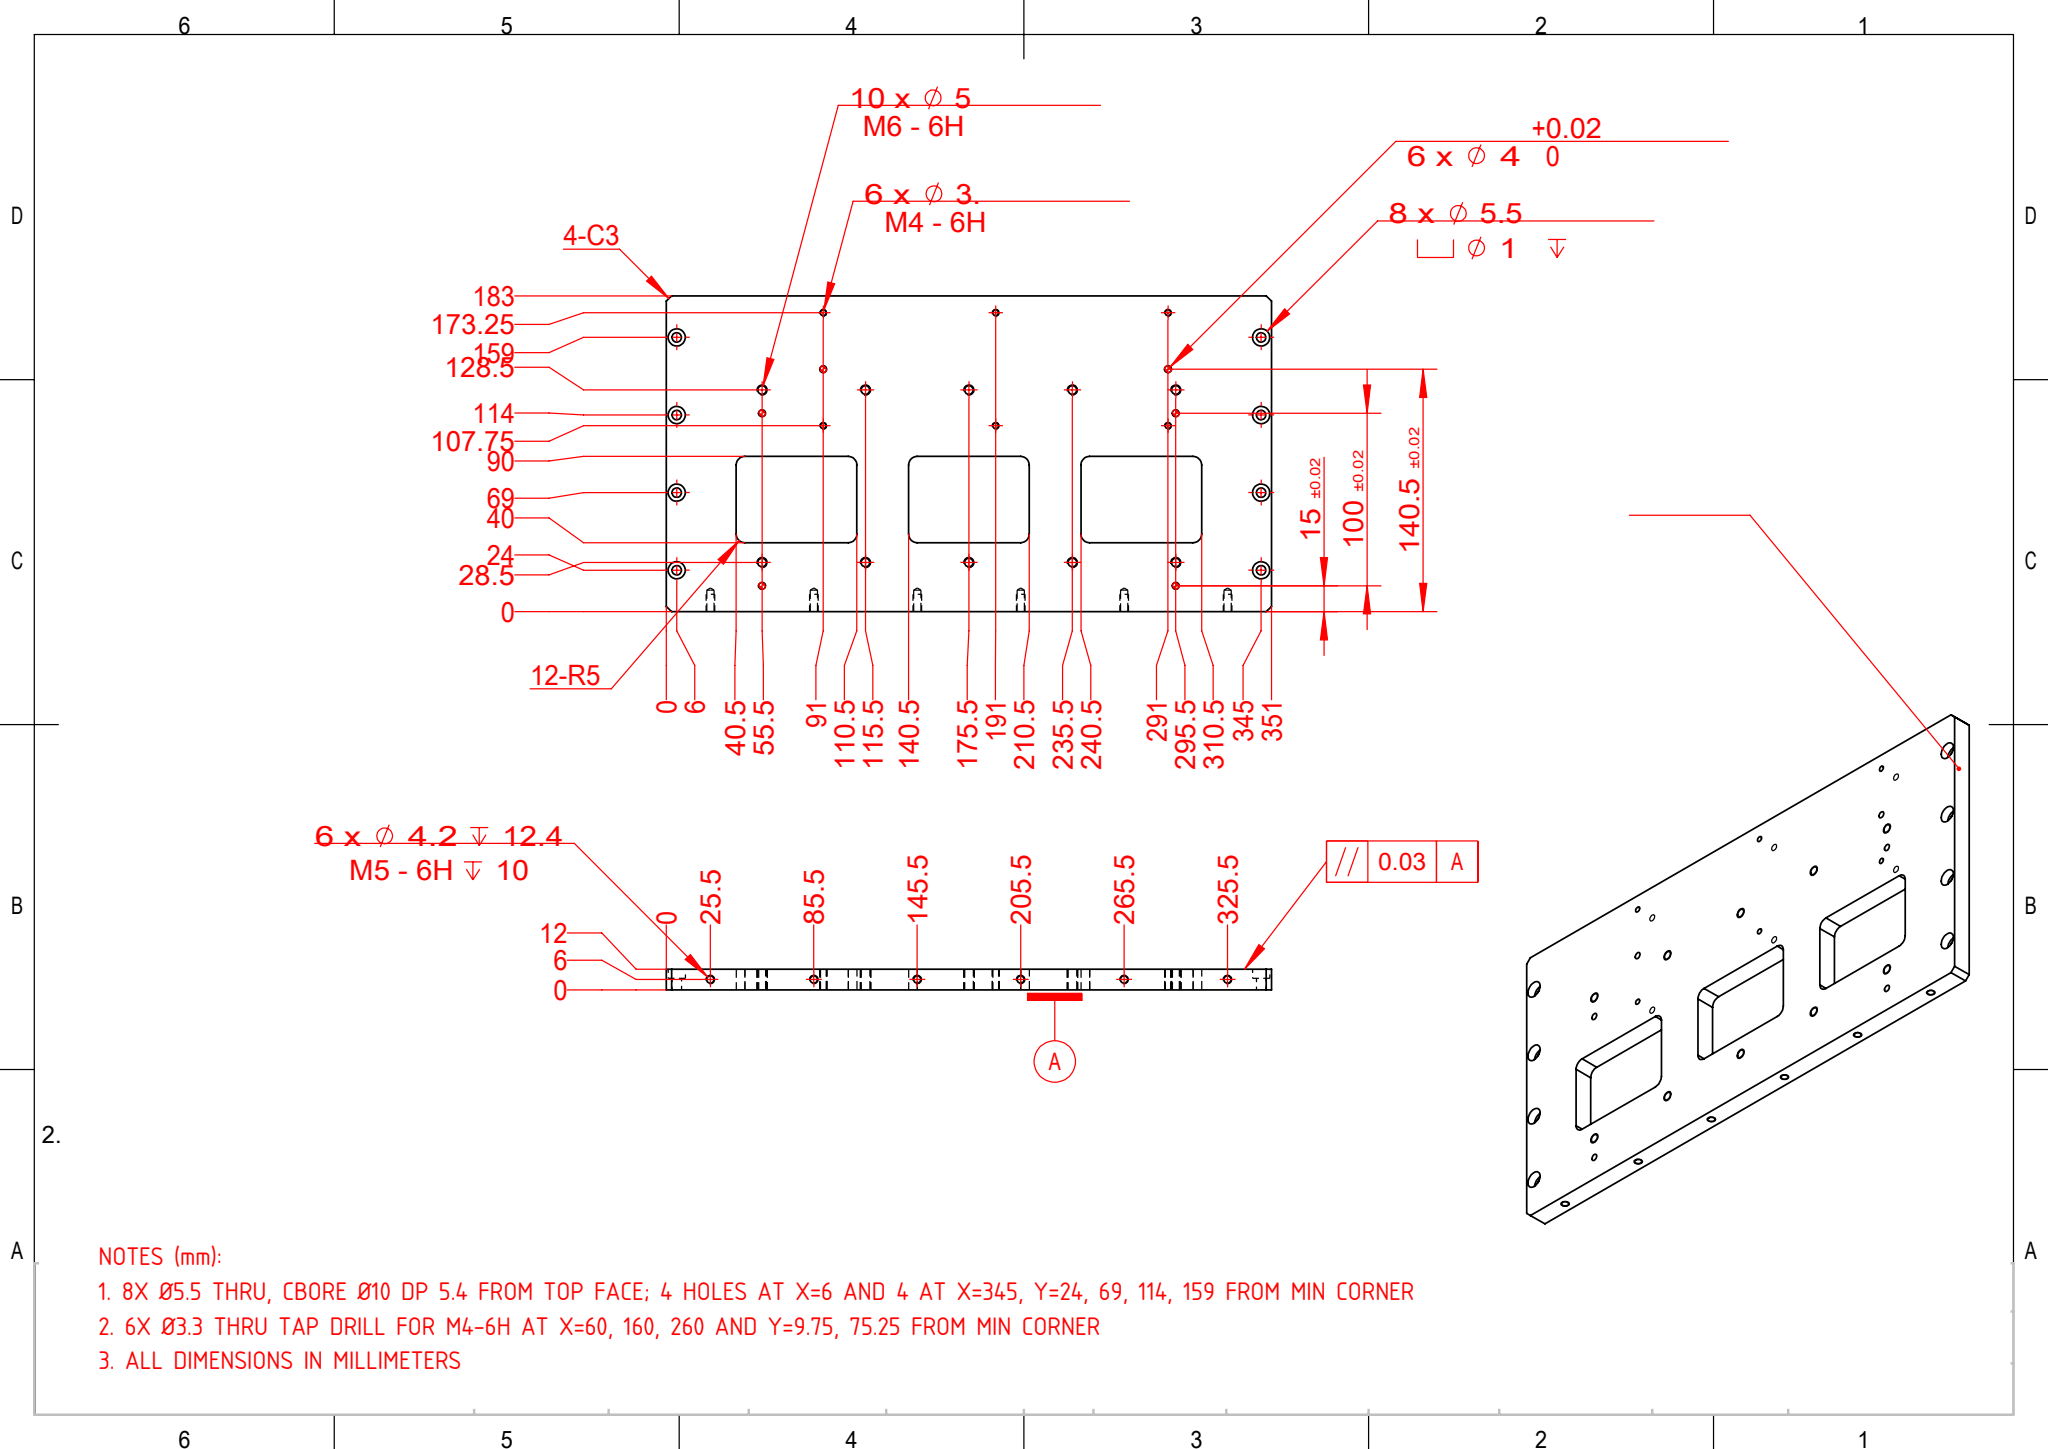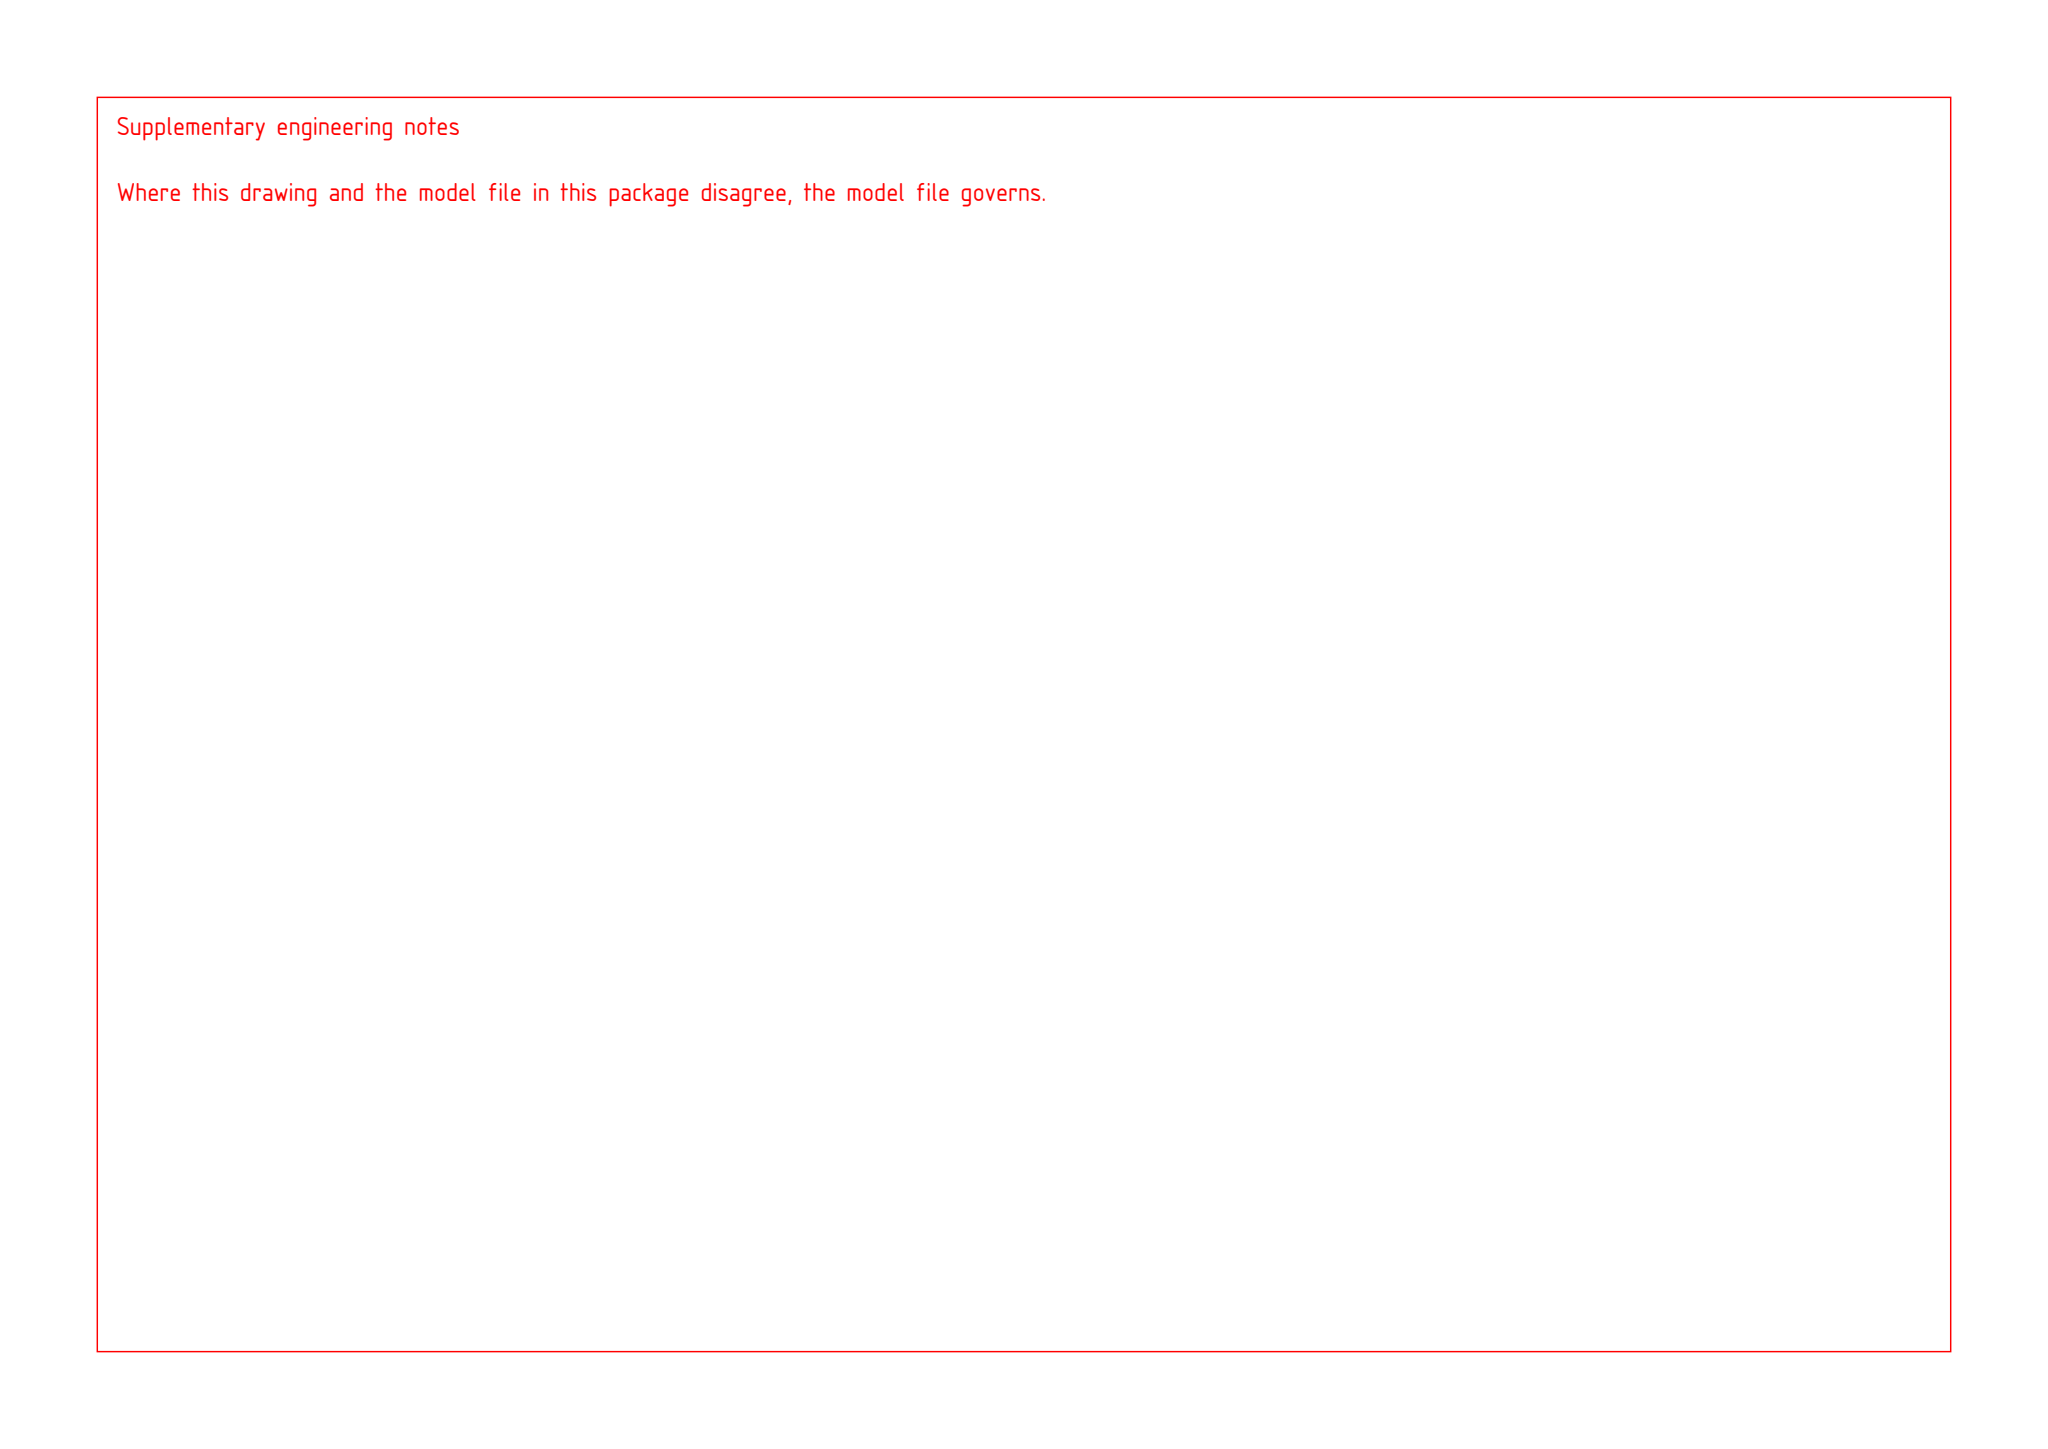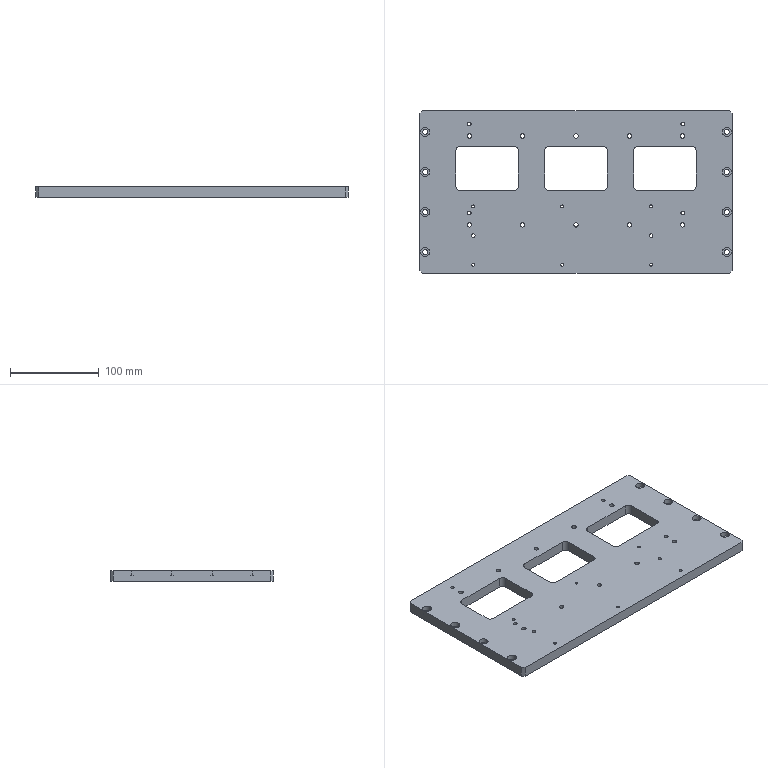Part | SolidWorks | mm | 1 solid | 142 faces | box 351 x 183 x 12 mm | volume 635763 mm3 | cylinder 100 | plane 30 | cone 12 | commonest cylinder face diameters 10 x28 5 x20 5.5 x16 4 x12 3.3 x12 4.2 x12
Drawing notes:
8X Ø5.5 THRU, CBORE Ø10 DP 5.4 FROM TOP FACE; 4 HOLES AT X=6 AND 4 AT X=345, Y=24, 69, 114, 159 FROM MIN CORNER | from the solid: cylinders [5.5,z,(6.0/345.0, 24/69/114/159),6.6] and [10.0,z,same positions,5.4]
6X Ø3.3 THRU TAP DRILL FOR M4-6H AT X=60, 160, 260 AND Y=9.75, 75.25 FROM MIN CORNER | from the solid: cylinders [3.3,z,(60/160/260, 9.75/75.25),12.0]
ALL DIMENSIONS IN MILLIMETERS | from the solid: STEP model facts stated in mm; bbox_xyz 351.0 x 183.0 x 12.0
build123d program:
from build123d import *

# Parameters (mm, degrees)
SKETCH1_W                                       = 351
SKETCH1_H                                       = 183
BOSS_EXTRUDE1_DEPTH                             = 12
SKETCH2_W                                       = 70
SKETCH2_H                                       = 50
CUT_EXTRUDE1_DEPTH                              = 199.284
LPATTERN1_COUNT                                 = 3
LPATTERN1_PITCH                                 = 100
FILLET1_R                                       = 5
M6_TAPPED_HOLE1_D                               = 5
SIZE_MM_DOWEL_PIN_HOLE1_D                       = 4
M5_HEX_SOCKET_HEAD_CAP_SCREW_CBORE2_D           = 5.5
M5_HEX_SOCKET_HEAD_CAP_SCREW_CBORE2_CBORE_D     = 10
M5_HEX_SOCKET_HEAD_CAP_SCREW_CBORE2_CBORE_DEPTH = 5.4
M5_TAPPED_HOLE1_D                               = 4.2
M5_TAPPED_HOLE1_DEPTH                           = 12.4
M5_TAPPED_HOLE1_TIP                             = 1.262
CHAMFER1_SIZE                                   = 3
M4_TAPPED_HOLE1_D                               = 3.3
SIZE_MM_DOWEL_PIN_HOLE3_D                       = 4


with BuildPart() as part:
    # Sketch1 → Boss-Extrude1 (new body)
    with BuildSketch(Plane.XY):
        Rectangle(SKETCH1_W, SKETCH1_H)
    extrude(amount=BOSS_EXTRUDE1_DEPTH)

    # Sketch2 → Cut-Extrude1 (cut, through all)
    with BuildSketch(Plane(origin=(0, 0, 0), x_dir=(-1, 0, 0), z_dir=(0, 0, -1))):
        with Locations((100, 26.5)):
            Rectangle(SKETCH2_W, SKETCH2_H)
    cut_extrude1 = extrude(amount=-CUT_EXTRUDE1_DEPTH, mode=Mode.SUBTRACT)

    # LPattern1: Cut-Extrude1 ×3
    with Locations(*[(i * LPATTERN1_PITCH, 0, 0) for i in range(1, LPATTERN1_COUNT)]):
        add(cut_extrude1, mode=Mode.SUBTRACT)

    # Fillet1
    fillet1_edges = [part.edges().sort_by_distance(p)[0] for p in [
        (-135, 51.5, 6),
        (-135, 1.5, 6),
        (-65, 1.5, 6),
        (-65, 51.5, 6),
        (-35, 51.5, 6),
        (-35, 1.5, 6),
        (35, 1.5, 6),
        (35, 51.5, 6),
        (65, 51.5, 6),
        (65, 1.5, 6),
        (135, 1.5, 6),
        (135, 51.5, 6),
    ]]
    fillet(fillet1_edges, radius=FILLET1_R)

    # M6 Tapped Hole1 (through all)
    with Locations(Plane.XY.offset(12)):
        with Locations((120, -37), (60, -37), (0, -37), (-60, -37), (-120, -37), (120, 63), (60, 63), (0, 63), (-60, 63), (-120, 63)):
            Hole(M6_TAPPED_HOLE1_D / 2)

    # Size mm Dowel Pin Hole1 (through all)
    with Locations(Plane.XY.offset(12)):
        with Locations((120, -23.5), (-120, -23.5), (120, 76.5), (-120, 76.5)):
            Hole(SIZE_MM_DOWEL_PIN_HOLE1_D / 2)

    # M5 Hex Socket Head Cap Screw CBORE2 (through all)
    with Locations(Plane.XY.offset(12)):
        with Locations((169.5, -67.5), (169.5, -22.5), (169.5, 22.5), (169.5, 67.5)):
            m5_hex_socket_head_cap_screw_cbore2 = CounterBoreHole(M5_HEX_SOCKET_HEAD_CAP_SCREW_CBORE2_D / 2, M5_HEX_SOCKET_HEAD_CAP_SCREW_CBORE2_CBORE_D / 2, M5_HEX_SOCKET_HEAD_CAP_SCREW_CBORE2_CBORE_DEPTH)

    # Mirror1: M5 Hex Socket Head Cap Screw CBORE2 across plane
    add(m5_hex_socket_head_cap_screw_cbore2.mirror(Plane(origin=(0, 0, 0), x_dir=(0, 0, 1), z_dir=(1, 0, 0))), mode=Mode.SUBTRACT)

    # M5 Tapped Hole1
    with Locations(Plane(origin=(0, 91.5, 0), x_dir=(1, 0, 0), z_dir=(0, 1, 0))):
        with Locations((150, -6), (90, -6), (30, -6), (-90, -6), (-150, -6), (-30, -6)):
            Hole(M5_TAPPED_HOLE1_D / 2, depth=M5_TAPPED_HOLE1_DEPTH)
            with Locations((0, 0, -(M5_TAPPED_HOLE1_DEPTH + M5_TAPPED_HOLE1_TIP / 2))):  # 118° drill point
                Cone(0, M5_TAPPED_HOLE1_D / 2, M5_TAPPED_HOLE1_TIP, mode=Mode.SUBTRACT)

    # Chamfer1
    chamfer1_edges = [part.edges().sort_by_distance(p)[0] for p in [
        (175.5, -91.5, 6),
        (-175.5, -91.5, 6),
        (-175.5, 91.5, 6),
        (175.5, 91.5, 6),
    ]]
    chamfer(chamfer1_edges, length=CHAMFER1_SIZE)

    # M4 Tapped Hole1 (through all)
    with Locations(Plane(origin=(0, 0, 0), x_dir=(-1, 0, 0), z_dir=(0, 0, -1))):
        with Locations((115.5, -81.75), (115.5, -16.25), (15.5, -16.25), (15.5, -81.75), (-84.5, -81.75), (-84.5, -16.25)):
            Hole(M4_TAPPED_HOLE1_D / 2)

    # Size mm Dowel Pin Hole3 (through all)
    with Locations(Plane.XY.offset(12)):
        with Locations((-115.5, -49), (84.5, -49)):
            Hole(SIZE_MM_DOWEL_PIN_HOLE3_D / 2)


solid = part.part